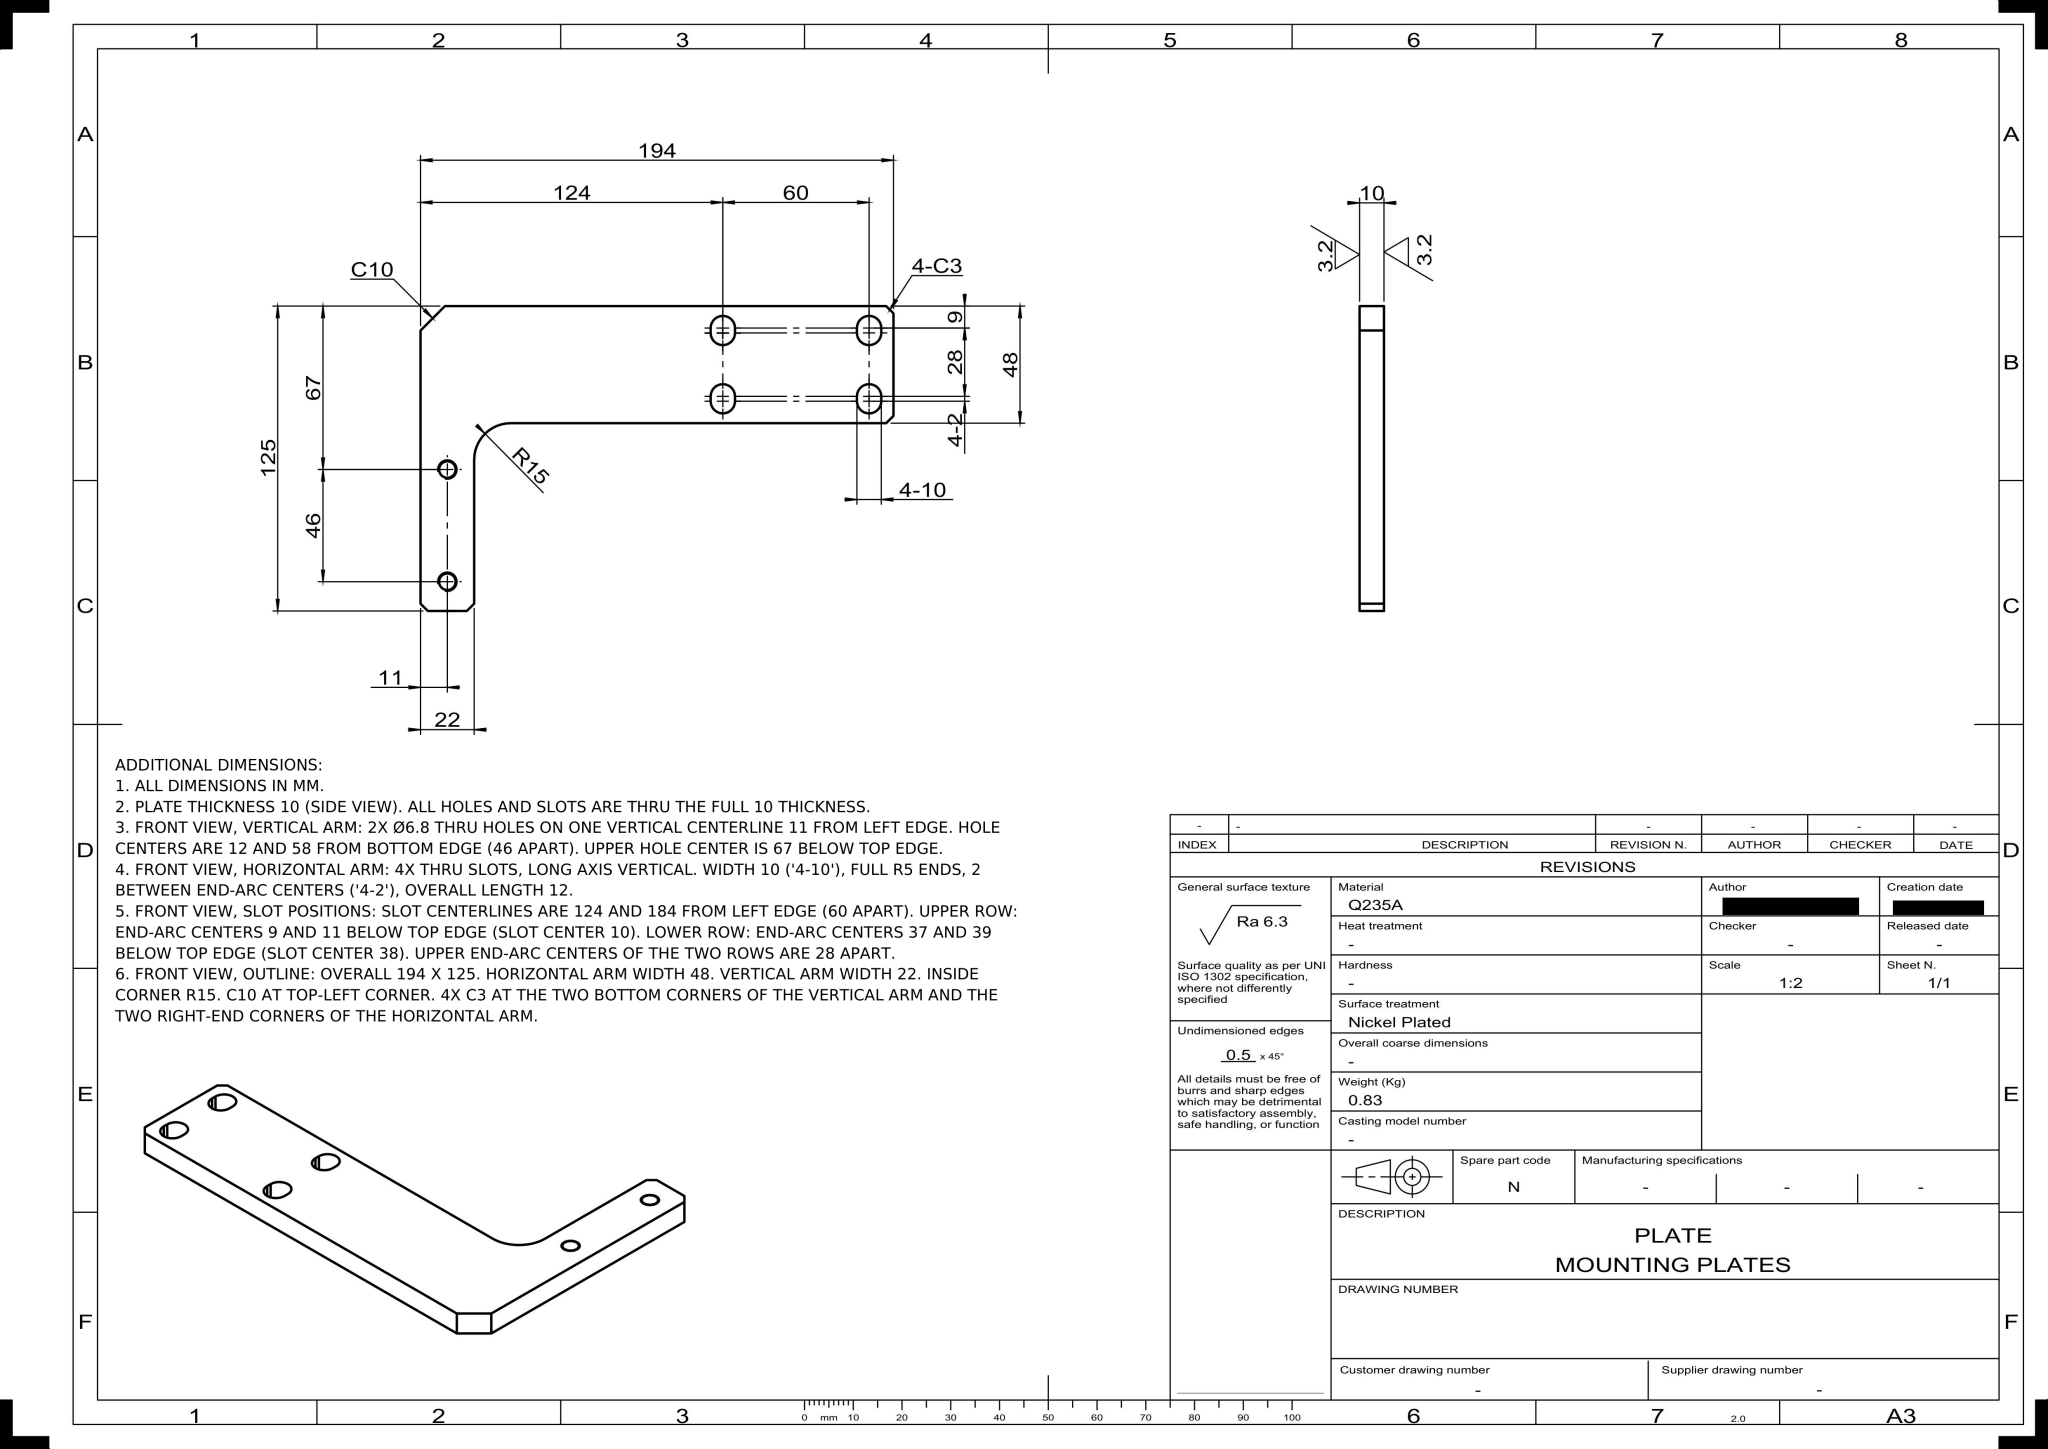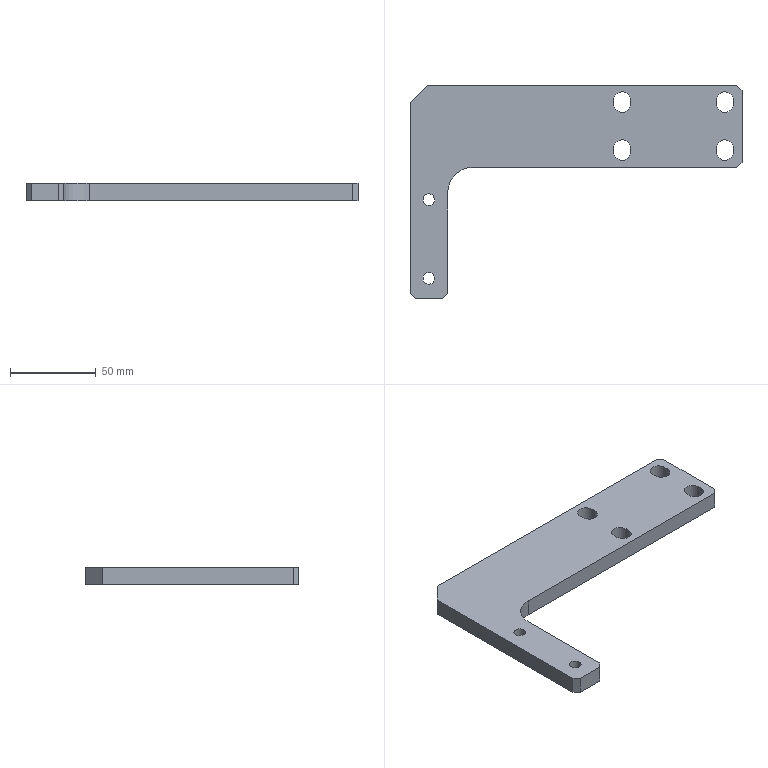Part | NX | mm | 1 solid | 32 faces | box 194 x 125 x 10 mm | volume 105195 mm3 | plane 21 | cylinder 11 | commonest cylinder face diameters 10 x8 6.8 x2 30 x1
STEP:
#1=CARTESIAN_POINT('',(0.,0.,0.));
#2=DIRECTION('',(0.,0.,1.));
#3=DIRECTION('',(1.,0.,0.));
#4=AXIS2_PLACEMENT_3D('',#1,#2,#3);
#5=(LENGTH_UNIT()NAMED_UNIT(*)SI_UNIT(.MILLI.,.METRE.));
#6=UNCERTAINTY_MEASURE_WITH_UNIT(LENGTH_MEASURE(0.00002),#5,'','');
#7=(NAMED_UNIT(*)PLANE_ANGLE_UNIT()SI_UNIT($,.RADIAN.));
#8=PLANE_ANGLE_MEASURE_WITH_UNIT(PLANE_ANGLE_MEASURE(0.01745),#7);
#9=DIMENSIONAL_EXPONENTS(0.,0.,0.,0.,0.,0.,0.);
#10=(CONVERSION_BASED_UNIT('',#8)NAMED_UNIT(#9)PLANE_ANGLE_UNIT());
#11=(NAMED_UNIT(*)SI_UNIT($,.STERADIAN.)SOLID_ANGLE_UNIT());
#12=(GEOMETRIC_REPRESENTATION_CONTEXT(3)GLOBAL_UNCERTAINTY_ASSIGNED_CONTEXT((#6))GLOBAL_UNIT_ASSIGNED_CONTEXT((#5,#10,#11))REPRESENTATION_CONTEXT('',''));
#13=SHAPE_REPRESENTATION('',(#4),#12);
#14=CARTESIAN_POINT('',(179.,-11.,0.));
#15=VERTEX_POINT('',#14);
#16=CARTESIAN_POINT('',(179.,-9.,0.));
#17=VERTEX_POINT('',#16);
#18=CARTESIAN_POINT('',(179.,-11.,0.));
#19=DIRECTION('',(0.,1.,0.));
#20=VECTOR('',#19,1.);
#21=LINE('',#18,#20);
#22=EDGE_CURVE('',#15,#17,#21,.T.);
#23=ORIENTED_EDGE('',*,*,#22,.T.);
#24=CARTESIAN_POINT('',(179.,-9.,10.));
#25=VERTEX_POINT('',#24);
#26=CARTESIAN_POINT('',(179.,-9.,10.));
#27=DIRECTION('',(0.,0.,-1.));
#28=VECTOR('',#27,1.);
#29=LINE('',#26,#28);
#30=EDGE_CURVE('',#25,#17,#29,.T.);
#31=ORIENTED_EDGE('',*,*,#30,.F.);
#32=CARTESIAN_POINT('',(179.,-11.,10.));
#33=VERTEX_POINT('',#32);
#34=CARTESIAN_POINT('',(179.,-11.,10.));
#35=DIRECTION('',(0.,1.,0.));
#36=VECTOR('',#35,1.);
#37=LINE('',#34,#36);
#38=EDGE_CURVE('',#33,#25,#37,.T.);
#39=ORIENTED_EDGE('',*,*,#38,.F.);
#40=CARTESIAN_POINT('',(179.,-11.,10.));
#41=DIRECTION('',(0.,0.,-1.));
#42=VECTOR('',#41,1.);
#43=LINE('',#40,#42);
#44=EDGE_CURVE('',#33,#15,#43,.T.);
#45=ORIENTED_EDGE('',*,*,#44,.T.);
#46=EDGE_LOOP('',(#23,#31,#39,#45));
#47=FACE_OUTER_BOUND('',#46,.T.);
#48=CARTESIAN_POINT('',(179.,-11.,10.));
#49=DIRECTION('',(-1.,0.,0.));
#50=DIRECTION('',(0.,0.,1.));
#51=AXIS2_PLACEMENT_3D('',#48,#49,#50);
#52=PLANE('',#51);
#53=ADVANCED_FACE('',(#47),#52,.F.);
#54=CARTESIAN_POINT('',(189.,-9.,0.));
#55=VERTEX_POINT('',#54);
#56=CARTESIAN_POINT('',(184.,-9.,0.));
#57=DIRECTION('',(0.,0.,-1.));
#58=DIRECTION('',(1.,0.,0.));
#59=AXIS2_PLACEMENT_3D('',#56,#57,#58);
#60=CIRCLE('',#59,5.);
#61=EDGE_CURVE('',#17,#55,#60,.T.);
#62=ORIENTED_EDGE('',*,*,#61,.T.);
#63=CARTESIAN_POINT('',(189.,-9.,10.));
#64=VERTEX_POINT('',#63);
#65=CARTESIAN_POINT('',(189.,-9.,10.));
#66=DIRECTION('',(0.,0.,-1.));
#67=VECTOR('',#66,1.);
#68=LINE('',#65,#67);
#69=EDGE_CURVE('',#64,#55,#68,.T.);
#70=ORIENTED_EDGE('',*,*,#69,.F.);
#71=CARTESIAN_POINT('',(184.,-9.,10.));
#72=DIRECTION('',(0.,0.,-1.));
#73=DIRECTION('',(1.,0.,0.));
#74=AXIS2_PLACEMENT_3D('',#71,#72,#73);
#75=CIRCLE('',#74,5.);
#76=EDGE_CURVE('',#25,#64,#75,.T.);
#77=ORIENTED_EDGE('',*,*,#76,.F.);
#78=ORIENTED_EDGE('',*,*,#30,.T.);
#79=EDGE_LOOP('',(#62,#70,#77,#78));
#80=FACE_OUTER_BOUND('',#79,.T.);
#81=CARTESIAN_POINT('',(184.,-9.,10.));
#82=DIRECTION('',(0.,0.,-1.));
#83=DIRECTION('',(-1.,0.,0.));
#84=AXIS2_PLACEMENT_3D('',#81,#82,#83);
#85=CYLINDRICAL_SURFACE('',#84,5.);
#86=ADVANCED_FACE('',(#80),#85,.F.);
#87=CARTESIAN_POINT('',(189.,-11.,0.));
#88=VERTEX_POINT('',#87);
#89=CARTESIAN_POINT('',(189.,-9.,0.));
#90=DIRECTION('',(0.,-1.,0.));
#91=VECTOR('',#90,1.);
#92=LINE('',#89,#91);
#93=EDGE_CURVE('',#55,#88,#92,.T.);
#94=ORIENTED_EDGE('',*,*,#93,.T.);
#95=CARTESIAN_POINT('',(189.,-11.,10.));
#96=VERTEX_POINT('',#95);
#97=CARTESIAN_POINT('',(189.,-11.,10.));
#98=DIRECTION('',(0.,0.,-1.));
#99=VECTOR('',#98,1.);
#100=LINE('',#97,#99);
#101=EDGE_CURVE('',#96,#88,#100,.T.);
#102=ORIENTED_EDGE('',*,*,#101,.F.);
#103=CARTESIAN_POINT('',(189.,-9.,10.));
#104=DIRECTION('',(0.,-1.,0.));
#105=VECTOR('',#104,1.);
#106=LINE('',#103,#105);
#107=EDGE_CURVE('',#64,#96,#106,.T.);
#108=ORIENTED_EDGE('',*,*,#107,.F.);
#109=ORIENTED_EDGE('',*,*,#69,.T.);
#110=EDGE_LOOP('',(#94,#102,#108,#109));
#111=FACE_OUTER_BOUND('',#110,.T.);
#112=CARTESIAN_POINT('',(189.,-9.,10.));
#113=DIRECTION('',(1.,0.,0.));
#114=DIRECTION('',(0.,0.,-1.));
#115=AXIS2_PLACEMENT_3D('',#112,#113,#114);
#116=PLANE('',#115);
#117=ADVANCED_FACE('',(#111),#116,.F.);
#118=CARTESIAN_POINT('',(179.,-39.,0.));
#119=VERTEX_POINT('',#118);
#120=CARTESIAN_POINT('',(179.,-37.,0.));
#121=VERTEX_POINT('',#120);
#122=CARTESIAN_POINT('',(179.,-39.,0.));
#123=DIRECTION('',(0.,1.,0.));
#124=VECTOR('',#123,1.);
#125=LINE('',#122,#124);
#126=EDGE_CURVE('',#119,#121,#125,.T.);
#127=ORIENTED_EDGE('',*,*,#126,.T.);
#128=CARTESIAN_POINT('',(179.,-37.,10.));
#129=VERTEX_POINT('',#128);
#130=CARTESIAN_POINT('',(179.,-37.,10.));
#131=DIRECTION('',(0.,0.,-1.));
#132=VECTOR('',#131,1.);
#133=LINE('',#130,#132);
#134=EDGE_CURVE('',#129,#121,#133,.T.);
#135=ORIENTED_EDGE('',*,*,#134,.F.);
#136=CARTESIAN_POINT('',(179.,-39.,10.));
#137=VERTEX_POINT('',#136);
#138=CARTESIAN_POINT('',(179.,-39.,10.));
#139=DIRECTION('',(0.,1.,0.));
#140=VECTOR('',#139,1.);
#141=LINE('',#138,#140);
#142=EDGE_CURVE('',#137,#129,#141,.T.);
#143=ORIENTED_EDGE('',*,*,#142,.F.);
#144=CARTESIAN_POINT('',(179.,-39.,10.));
#145=DIRECTION('',(0.,0.,-1.));
#146=VECTOR('',#145,1.);
#147=LINE('',#144,#146);
#148=EDGE_CURVE('',#137,#119,#147,.T.);
#149=ORIENTED_EDGE('',*,*,#148,.T.);
#150=EDGE_LOOP('',(#127,#135,#143,#149));
#151=FACE_OUTER_BOUND('',#150,.T.);
#152=CARTESIAN_POINT('',(179.,-39.,10.));
#153=DIRECTION('',(-1.,0.,0.));
#154=DIRECTION('',(0.,0.,1.));
#155=AXIS2_PLACEMENT_3D('',#152,#153,#154);
#156=PLANE('',#155);
#157=ADVANCED_FACE('',(#151),#156,.F.);
#158=CARTESIAN_POINT('',(189.,-37.,0.));
#159=VERTEX_POINT('',#158);
#160=CARTESIAN_POINT('',(184.,-37.,0.));
#161=DIRECTION('',(0.,0.,-1.));
#162=DIRECTION('',(1.,0.,0.));
#163=AXIS2_PLACEMENT_3D('',#160,#161,#162);
#164=CIRCLE('',#163,5.);
#165=EDGE_CURVE('',#121,#159,#164,.T.);
#166=ORIENTED_EDGE('',*,*,#165,.T.);
#167=CARTESIAN_POINT('',(189.,-37.,10.));
#168=VERTEX_POINT('',#167);
#169=CARTESIAN_POINT('',(189.,-37.,10.));
#170=DIRECTION('',(0.,0.,-1.));
#171=VECTOR('',#170,1.);
#172=LINE('',#169,#171);
#173=EDGE_CURVE('',#168,#159,#172,.T.);
#174=ORIENTED_EDGE('',*,*,#173,.F.);
#175=CARTESIAN_POINT('',(184.,-37.,10.));
#176=DIRECTION('',(0.,0.,-1.));
#177=DIRECTION('',(1.,0.,0.));
#178=AXIS2_PLACEMENT_3D('',#175,#176,#177);
#179=CIRCLE('',#178,5.);
#180=EDGE_CURVE('',#129,#168,#179,.T.);
#181=ORIENTED_EDGE('',*,*,#180,.F.);
#182=ORIENTED_EDGE('',*,*,#134,.T.);
#183=EDGE_LOOP('',(#166,#174,#181,#182));
#184=FACE_OUTER_BOUND('',#183,.T.);
#185=CARTESIAN_POINT('',(184.,-37.,10.));
#186=DIRECTION('',(0.,0.,-1.));
#187=DIRECTION('',(-1.,0.,0.));
#188=AXIS2_PLACEMENT_3D('',#185,#186,#187);
#189=CYLINDRICAL_SURFACE('',#188,5.);
#190=ADVANCED_FACE('',(#184),#189,.F.);
#191=CARTESIAN_POINT('',(189.,-39.,0.));
#192=VERTEX_POINT('',#191);
#193=CARTESIAN_POINT('',(189.,-37.,0.));
#194=DIRECTION('',(0.,-1.,0.));
#195=VECTOR('',#194,1.);
#196=LINE('',#193,#195);
#197=EDGE_CURVE('',#159,#192,#196,.T.);
#198=ORIENTED_EDGE('',*,*,#197,.T.);
#199=CARTESIAN_POINT('',(189.,-39.,10.));
#200=VERTEX_POINT('',#199);
#201=CARTESIAN_POINT('',(189.,-39.,10.));
#202=DIRECTION('',(0.,0.,-1.));
#203=VECTOR('',#202,1.);
#204=LINE('',#201,#203);
#205=EDGE_CURVE('',#200,#192,#204,.T.);
#206=ORIENTED_EDGE('',*,*,#205,.F.);
#207=CARTESIAN_POINT('',(189.,-37.,10.));
#208=DIRECTION('',(0.,-1.,0.));
#209=VECTOR('',#208,1.);
#210=LINE('',#207,#209);
#211=EDGE_CURVE('',#168,#200,#210,.T.);
#212=ORIENTED_EDGE('',*,*,#211,.F.);
#213=ORIENTED_EDGE('',*,*,#173,.T.);
#214=EDGE_LOOP('',(#198,#206,#212,#213));
#215=FACE_OUTER_BOUND('',#214,.T.);
#216=CARTESIAN_POINT('',(189.,-37.,10.));
#217=DIRECTION('',(1.,0.,0.));
#218=DIRECTION('',(0.,0.,-1.));
#219=AXIS2_PLACEMENT_3D('',#216,#217,#218);
#220=PLANE('',#219);
#221=ADVANCED_FACE('',(#215),#220,.F.);
#222=CARTESIAN_POINT('',(119.,-11.,0.));
#223=VERTEX_POINT('',#222);
#224=CARTESIAN_POINT('',(119.,-9.,0.));
#225=VERTEX_POINT('',#224);
#226=CARTESIAN_POINT('',(119.,-11.,0.));
#227=DIRECTION('',(0.,1.,0.));
#228=VECTOR('',#227,1.);
#229=LINE('',#226,#228);
#230=EDGE_CURVE('',#223,#225,#229,.T.);
#231=ORIENTED_EDGE('',*,*,#230,.T.);
#232=CARTESIAN_POINT('',(119.,-9.,10.));
#233=VERTEX_POINT('',#232);
#234=CARTESIAN_POINT('',(119.,-9.,10.));
#235=DIRECTION('',(0.,0.,-1.));
#236=VECTOR('',#235,1.);
#237=LINE('',#234,#236);
#238=EDGE_CURVE('',#233,#225,#237,.T.);
#239=ORIENTED_EDGE('',*,*,#238,.F.);
#240=CARTESIAN_POINT('',(119.,-11.,10.));
#241=VERTEX_POINT('',#240);
#242=CARTESIAN_POINT('',(119.,-11.,10.));
#243=DIRECTION('',(0.,1.,0.));
#244=VECTOR('',#243,1.);
#245=LINE('',#242,#244);
#246=EDGE_CURVE('',#241,#233,#245,.T.);
#247=ORIENTED_EDGE('',*,*,#246,.F.);
#248=CARTESIAN_POINT('',(119.,-11.,10.));
#249=DIRECTION('',(0.,0.,-1.));
#250=VECTOR('',#249,1.);
#251=LINE('',#248,#250);
#252=EDGE_CURVE('',#241,#223,#251,.T.);
#253=ORIENTED_EDGE('',*,*,#252,.T.);
#254=EDGE_LOOP('',(#231,#239,#247,#253));
#255=FACE_OUTER_BOUND('',#254,.T.);
#256=CARTESIAN_POINT('',(119.,-11.,10.));
#257=DIRECTION('',(-1.,0.,0.));
#258=DIRECTION('',(0.,0.,1.));
#259=AXIS2_PLACEMENT_3D('',#256,#257,#258);
#260=PLANE('',#259);
#261=ADVANCED_FACE('',(#255),#260,.F.);
#262=CARTESIAN_POINT('',(129.,-9.,0.));
#263=VERTEX_POINT('',#262);
#264=CARTESIAN_POINT('',(124.,-9.,0.));
#265=DIRECTION('',(0.,0.,-1.));
#266=DIRECTION('',(1.,0.,0.));
#267=AXIS2_PLACEMENT_3D('',#264,#265,#266);
#268=CIRCLE('',#267,5.);
#269=EDGE_CURVE('',#225,#263,#268,.T.);
#270=ORIENTED_EDGE('',*,*,#269,.T.);
#271=CARTESIAN_POINT('',(129.,-9.,10.));
#272=VERTEX_POINT('',#271);
#273=CARTESIAN_POINT('',(129.,-9.,10.));
#274=DIRECTION('',(0.,0.,-1.));
#275=VECTOR('',#274,1.);
#276=LINE('',#273,#275);
#277=EDGE_CURVE('',#272,#263,#276,.T.);
#278=ORIENTED_EDGE('',*,*,#277,.F.);
#279=CARTESIAN_POINT('',(124.,-9.,10.));
#280=DIRECTION('',(0.,0.,-1.));
#281=DIRECTION('',(1.,0.,0.));
#282=AXIS2_PLACEMENT_3D('',#279,#280,#281);
#283=CIRCLE('',#282,5.);
#284=EDGE_CURVE('',#233,#272,#283,.T.);
#285=ORIENTED_EDGE('',*,*,#284,.F.);
#286=ORIENTED_EDGE('',*,*,#238,.T.);
#287=EDGE_LOOP('',(#270,#278,#285,#286));
#288=FACE_OUTER_BOUND('',#287,.T.);
#289=CARTESIAN_POINT('',(124.,-9.,10.));
#290=DIRECTION('',(0.,0.,-1.));
#291=DIRECTION('',(-1.,0.,0.));
#292=AXIS2_PLACEMENT_3D('',#289,#290,#291);
#293=CYLINDRICAL_SURFACE('',#292,5.);
#294=ADVANCED_FACE('',(#288),#293,.F.);
#295=CARTESIAN_POINT('',(129.,-11.,0.));
#296=VERTEX_POINT('',#295);
#297=CARTESIAN_POINT('',(129.,-9.,0.));
#298=DIRECTION('',(0.,-1.,0.));
#299=VECTOR('',#298,1.);
#300=LINE('',#297,#299);
#301=EDGE_CURVE('',#263,#296,#300,.T.);
#302=ORIENTED_EDGE('',*,*,#301,.T.);
#303=CARTESIAN_POINT('',(129.,-11.,10.));
#304=VERTEX_POINT('',#303);
#305=CARTESIAN_POINT('',(129.,-11.,10.));
#306=DIRECTION('',(0.,0.,-1.));
#307=VECTOR('',#306,1.);
#308=LINE('',#305,#307);
#309=EDGE_CURVE('',#304,#296,#308,.T.);
#310=ORIENTED_EDGE('',*,*,#309,.F.);
#311=CARTESIAN_POINT('',(129.,-9.,10.));
#312=DIRECTION('',(0.,-1.,0.));
#313=VECTOR('',#312,1.);
#314=LINE('',#311,#313);
#315=EDGE_CURVE('',#272,#304,#314,.T.);
#316=ORIENTED_EDGE('',*,*,#315,.F.);
#317=ORIENTED_EDGE('',*,*,#277,.T.);
#318=EDGE_LOOP('',(#302,#310,#316,#317));
#319=FACE_OUTER_BOUND('',#318,.T.);
#320=CARTESIAN_POINT('',(129.,-9.,10.));
#321=DIRECTION('',(1.,0.,0.));
#322=DIRECTION('',(0.,0.,-1.));
#323=AXIS2_PLACEMENT_3D('',#320,#321,#322);
#324=PLANE('',#323);
#325=ADVANCED_FACE('',(#319),#324,.F.);
#326=CARTESIAN_POINT('',(119.,-39.,0.));
#327=VERTEX_POINT('',#326);
#328=CARTESIAN_POINT('',(119.,-37.,0.));
#329=VERTEX_POINT('',#328);
#330=CARTESIAN_POINT('',(119.,-39.,0.));
#331=DIRECTION('',(0.,1.,0.));
#332=VECTOR('',#331,1.);
#333=LINE('',#330,#332);
#334=EDGE_CURVE('',#327,#329,#333,.T.);
#335=ORIENTED_EDGE('',*,*,#334,.T.);
#336=CARTESIAN_POINT('',(119.,-37.,10.));
#337=VERTEX_POINT('',#336);
#338=CARTESIAN_POINT('',(119.,-37.,10.));
#339=DIRECTION('',(0.,0.,-1.));
#340=VECTOR('',#339,1.);
#341=LINE('',#338,#340);
#342=EDGE_CURVE('',#337,#329,#341,.T.);
#343=ORIENTED_EDGE('',*,*,#342,.F.);
#344=CARTESIAN_POINT('',(119.,-39.,10.));
#345=VERTEX_POINT('',#344);
#346=CARTESIAN_POINT('',(119.,-39.,10.));
#347=DIRECTION('',(0.,1.,0.));
#348=VECTOR('',#347,1.);
#349=LINE('',#346,#348);
#350=EDGE_CURVE('',#345,#337,#349,.T.);
#351=ORIENTED_EDGE('',*,*,#350,.F.);
#352=CARTESIAN_POINT('',(119.,-39.,10.));
#353=DIRECTION('',(0.,0.,-1.));
#354=VECTOR('',#353,1.);
#355=LINE('',#352,#354);
#356=EDGE_CURVE('',#345,#327,#355,.T.);
#357=ORIENTED_EDGE('',*,*,#356,.T.);
#358=EDGE_LOOP('',(#335,#343,#351,#357));
#359=FACE_OUTER_BOUND('',#358,.T.);
#360=CARTESIAN_POINT('',(119.,-39.,10.));
#361=DIRECTION('',(-1.,0.,0.));
#362=DIRECTION('',(0.,0.,1.));
#363=AXIS2_PLACEMENT_3D('',#360,#361,#362);
#364=PLANE('',#363);
#365=ADVANCED_FACE('',(#359),#364,.F.);
#366=CARTESIAN_POINT('',(129.,-37.,0.));
#367=VERTEX_POINT('',#366);
#368=CARTESIAN_POINT('',(124.,-37.,0.));
#369=DIRECTION('',(0.,0.,-1.));
#370=DIRECTION('',(1.,0.,0.));
#371=AXIS2_PLACEMENT_3D('',#368,#369,#370);
#372=CIRCLE('',#371,5.);
#373=EDGE_CURVE('',#329,#367,#372,.T.);
#374=ORIENTED_EDGE('',*,*,#373,.T.);
#375=CARTESIAN_POINT('',(129.,-37.,10.));
#376=VERTEX_POINT('',#375);
#377=CARTESIAN_POINT('',(129.,-37.,10.));
#378=DIRECTION('',(0.,0.,-1.));
#379=VECTOR('',#378,1.);
#380=LINE('',#377,#379);
#381=EDGE_CURVE('',#376,#367,#380,.T.);
#382=ORIENTED_EDGE('',*,*,#381,.F.);
#383=CARTESIAN_POINT('',(124.,-37.,10.));
#384=DIRECTION('',(0.,0.,-1.));
#385=DIRECTION('',(1.,0.,0.));
#386=AXIS2_PLACEMENT_3D('',#383,#384,#385);
#387=CIRCLE('',#386,5.);
#388=EDGE_CURVE('',#337,#376,#387,.T.);
#389=ORIENTED_EDGE('',*,*,#388,.F.);
#390=ORIENTED_EDGE('',*,*,#342,.T.);
#391=EDGE_LOOP('',(#374,#382,#389,#390));
#392=FACE_OUTER_BOUND('',#391,.T.);
#393=CARTESIAN_POINT('',(124.,-37.,10.));
#394=DIRECTION('',(0.,0.,-1.));
#395=DIRECTION('',(-1.,0.,0.));
#396=AXIS2_PLACEMENT_3D('',#393,#394,#395);
#397=CYLINDRICAL_SURFACE('',#396,5.);
#398=ADVANCED_FACE('',(#392),#397,.F.);
#399=CARTESIAN_POINT('',(129.,-39.,0.));
#400=VERTEX_POINT('',#399);
#401=CARTESIAN_POINT('',(129.,-37.,0.));
#402=DIRECTION('',(0.,-1.,0.));
#403=VECTOR('',#402,1.);
#404=LINE('',#401,#403);
#405=EDGE_CURVE('',#367,#400,#404,.T.);
#406=ORIENTED_EDGE('',*,*,#405,.T.);
#407=CARTESIAN_POINT('',(129.,-39.,10.));
#408=VERTEX_POINT('',#407);
#409=CARTESIAN_POINT('',(129.,-39.,10.));
#410=DIRECTION('',(0.,0.,-1.));
#411=VECTOR('',#410,1.);
#412=LINE('',#409,#411);
#413=EDGE_CURVE('',#408,#400,#412,.T.);
#414=ORIENTED_EDGE('',*,*,#413,.F.);
#415=CARTESIAN_POINT('',(129.,-37.,10.));
#416=DIRECTION('',(0.,-1.,0.));
#417=VECTOR('',#416,1.);
#418=LINE('',#415,#417);
#419=EDGE_CURVE('',#376,#408,#418,.T.);
#420=ORIENTED_EDGE('',*,*,#419,.F.);
#421=ORIENTED_EDGE('',*,*,#381,.T.);
#422=EDGE_LOOP('',(#406,#414,#420,#421));
#423=FACE_OUTER_BOUND('',#422,.T.);
#424=CARTESIAN_POINT('',(129.,-37.,10.));
#425=DIRECTION('',(1.,0.,0.));
#426=DIRECTION('',(0.,0.,-1.));
#427=AXIS2_PLACEMENT_3D('',#424,#425,#426);
#428=PLANE('',#427);
#429=ADVANCED_FACE('',(#423),#428,.F.);
#430=CARTESIAN_POINT('',(0.,-10.,0.));
#431=VERTEX_POINT('',#430);
#432=CARTESIAN_POINT('',(0.,-122.,0.));
#433=VERTEX_POINT('',#432);
#434=CARTESIAN_POINT('',(0.,0.,0.));
#435=DIRECTION('',(0.,-1.,0.));
#436=VECTOR('',#435,1.);
#437=LINE('',#434,#436);
#438=EDGE_CURVE('',#431,#433,#437,.T.);
#439=ORIENTED_EDGE('',*,*,#438,.T.);
#440=CARTESIAN_POINT('',(0.,-122.,10.));
#441=VERTEX_POINT('',#440);
#442=CARTESIAN_POINT('',(0.,-122.,10.));
#443=DIRECTION('',(0.,0.,1.));
#444=VECTOR('',#443,1.);
#445=LINE('',#442,#444);
#446=EDGE_CURVE('',#433,#441,#445,.T.);
#447=ORIENTED_EDGE('',*,*,#446,.T.);
#448=CARTESIAN_POINT('',(0.,-10.,10.));
#449=VERTEX_POINT('',#448);
#450=CARTESIAN_POINT('',(0.,0.,10.));
#451=DIRECTION('',(0.,-1.,0.));
#452=VECTOR('',#451,1.);
#453=LINE('',#450,#452);
#454=EDGE_CURVE('',#449,#441,#453,.T.);
#455=ORIENTED_EDGE('',*,*,#454,.F.);
#456=CARTESIAN_POINT('',(0.,-10.,10.));
#457=DIRECTION('',(0.,0.,-1.));
#458=VECTOR('',#457,1.);
#459=LINE('',#456,#458);
#460=EDGE_CURVE('',#449,#431,#459,.T.);
#461=ORIENTED_EDGE('',*,*,#460,.T.);
#462=EDGE_LOOP('',(#439,#447,#455,#461));
#463=FACE_OUTER_BOUND('',#462,.T.);
#464=CARTESIAN_POINT('',(0.,0.,10.));
#465=DIRECTION('',(1.,0.,0.));
#466=DIRECTION('',(0.,0.,-1.));
#467=AXIS2_PLACEMENT_3D('',#464,#465,#466);
#468=PLANE('',#467);
#469=ADVANCED_FACE('',(#463),#468,.F.);
#470=CARTESIAN_POINT('',(3.,-125.,0.));
#471=VERTEX_POINT('',#470);
#472=CARTESIAN_POINT('',(19.,-125.,0.));
#473=VERTEX_POINT('',#472);
#474=CARTESIAN_POINT('',(-0.,-125.,0.));
#475=DIRECTION('',(1.,0.,0.));
#476=VECTOR('',#475,1.);
#477=LINE('',#474,#476);
#478=EDGE_CURVE('',#471,#473,#477,.T.);
#479=ORIENTED_EDGE('',*,*,#478,.T.);
#480=CARTESIAN_POINT('',(19.,-125.,10.));
#481=VERTEX_POINT('',#480);
#482=CARTESIAN_POINT('',(19.,-125.,10.));
#483=DIRECTION('',(0.,0.,1.));
#484=VECTOR('',#483,1.);
#485=LINE('',#482,#484);
#486=EDGE_CURVE('',#473,#481,#485,.T.);
#487=ORIENTED_EDGE('',*,*,#486,.T.);
#488=CARTESIAN_POINT('',(3.,-125.,10.));
#489=VERTEX_POINT('',#488);
#490=CARTESIAN_POINT('',(-0.,-125.,10.));
#491=DIRECTION('',(1.,0.,0.));
#492=VECTOR('',#491,1.);
#493=LINE('',#490,#492);
#494=EDGE_CURVE('',#489,#481,#493,.T.);
#495=ORIENTED_EDGE('',*,*,#494,.F.);
#496=CARTESIAN_POINT('',(3.,-125.,10.));
#497=DIRECTION('',(0.,0.,-1.));
#498=VECTOR('',#497,1.);
#499=LINE('',#496,#498);
#500=EDGE_CURVE('',#489,#471,#499,.T.);
#501=ORIENTED_EDGE('',*,*,#500,.T.);
#502=EDGE_LOOP('',(#479,#487,#495,#501));
#503=FACE_OUTER_BOUND('',#502,.T.);
#504=CARTESIAN_POINT('',(-0.,-125.,10.));
#505=DIRECTION('',(0.,1.,0.));
#506=DIRECTION('',(0.,0.,1.));
#507=AXIS2_PLACEMENT_3D('',#504,#505,#506);
#508=PLANE('',#507);
#509=ADVANCED_FACE('',(#503),#508,.F.);
#510=CARTESIAN_POINT('',(22.,-122.,0.));
#511=VERTEX_POINT('',#510);
#512=CARTESIAN_POINT('',(22.,-63.,0.));
#513=VERTEX_POINT('',#512);
#514=CARTESIAN_POINT('',(22.,-125.,0.));
#515=DIRECTION('',(0.,1.,0.));
#516=VECTOR('',#515,1.);
#517=LINE('',#514,#516);
#518=EDGE_CURVE('',#511,#513,#517,.T.);
#519=ORIENTED_EDGE('',*,*,#518,.T.);
#520=CARTESIAN_POINT('',(22.,-63.,10.));
#521=VERTEX_POINT('',#520);
#522=CARTESIAN_POINT('',(22.,-63.,10.));
#523=DIRECTION('',(0.,0.,1.));
#524=VECTOR('',#523,1.);
#525=LINE('',#522,#524);
#526=EDGE_CURVE('',#513,#521,#525,.T.);
#527=ORIENTED_EDGE('',*,*,#526,.T.);
#528=CARTESIAN_POINT('',(22.,-122.,10.));
#529=VERTEX_POINT('',#528);
#530=CARTESIAN_POINT('',(22.,-125.,10.));
#531=DIRECTION('',(0.,1.,0.));
#532=VECTOR('',#531,1.);
#533=LINE('',#530,#532);
#534=EDGE_CURVE('',#529,#521,#533,.T.);
#535=ORIENTED_EDGE('',*,*,#534,.F.);
#536=CARTESIAN_POINT('',(22.,-122.,10.));
#537=DIRECTION('',(0.,0.,-1.));
#538=VECTOR('',#537,1.);
#539=LINE('',#536,#538);
#540=EDGE_CURVE('',#529,#511,#539,.T.);
#541=ORIENTED_EDGE('',*,*,#540,.T.);
#542=EDGE_LOOP('',(#519,#527,#535,#541));
#543=FACE_OUTER_BOUND('',#542,.T.);
#544=CARTESIAN_POINT('',(22.,-125.,10.));
#545=DIRECTION('',(-1.,0.,0.));
#546=DIRECTION('',(-0.,-1.,0.));
#547=AXIS2_PLACEMENT_3D('',#544,#545,#546);
#548=PLANE('',#547);
#549=ADVANCED_FACE('',(#543),#548,.F.);
#550=CARTESIAN_POINT('',(37.,-48.,10.));
#551=VERTEX_POINT('',#550);
#552=CARTESIAN_POINT('',(191.,-48.,10.));
#553=VERTEX_POINT('',#552);
#554=CARTESIAN_POINT('',(22.,-48.,10.));
#555=DIRECTION('',(1.,0.,0.));
#556=VECTOR('',#555,1.);
#557=LINE('',#554,#556);
#558=EDGE_CURVE('',#551,#553,#557,.T.);
#559=ORIENTED_EDGE('',*,*,#558,.F.);
#560=CARTESIAN_POINT('',(37.,-48.,0.));
#561=VERTEX_POINT('',#560);
#562=CARTESIAN_POINT('',(37.,-48.,0.));
#563=DIRECTION('',(0.,0.,-1.));
#564=VECTOR('',#563,1.);
#565=LINE('',#562,#564);
#566=EDGE_CURVE('',#551,#561,#565,.T.);
#567=ORIENTED_EDGE('',*,*,#566,.T.);
#568=CARTESIAN_POINT('',(191.,-48.,0.));
#569=VERTEX_POINT('',#568);
#570=CARTESIAN_POINT('',(22.,-48.,0.));
#571=DIRECTION('',(1.,0.,0.));
#572=VECTOR('',#571,1.);
#573=LINE('',#570,#572);
#574=EDGE_CURVE('',#561,#569,#573,.T.);
#575=ORIENTED_EDGE('',*,*,#574,.T.);
#576=CARTESIAN_POINT('',(191.,-48.,10.));
#577=DIRECTION('',(0.,0.,1.));
#578=VECTOR('',#577,1.);
#579=LINE('',#576,#578);
#580=EDGE_CURVE('',#569,#553,#579,.T.);
#581=ORIENTED_EDGE('',*,*,#580,.T.);
#582=EDGE_LOOP('',(#559,#567,#575,#581));
#583=FACE_OUTER_BOUND('',#582,.T.);
#584=CARTESIAN_POINT('',(22.,-48.,10.));
#585=DIRECTION('',(0.,1.,0.));
#586=DIRECTION('',(0.,0.,1.));
#587=AXIS2_PLACEMENT_3D('',#584,#585,#586);
#588=PLANE('',#587);
#589=ADVANCED_FACE('',(#583),#588,.F.);
#590=CARTESIAN_POINT('',(194.,-45.,10.));
#591=VERTEX_POINT('',#590);
#592=CARTESIAN_POINT('',(194.,-3.,10.));
#593=VERTEX_POINT('',#592);
#594=CARTESIAN_POINT('',(194.,-48.,10.));
#595=DIRECTION('',(0.,1.,0.));
#596=VECTOR('',#595,1.);
#597=LINE('',#594,#596);
#598=EDGE_CURVE('',#591,#593,#597,.T.);
#599=ORIENTED_EDGE('',*,*,#598,.F.);
#600=CARTESIAN_POINT('',(194.,-45.,0.));
#601=VERTEX_POINT('',#600);
#602=CARTESIAN_POINT('',(194.,-45.,10.));
#603=DIRECTION('',(0.,0.,-1.));
#604=VECTOR('',#603,1.);
#605=LINE('',#602,#604);
#606=EDGE_CURVE('',#591,#601,#605,.T.);
#607=ORIENTED_EDGE('',*,*,#606,.T.);
#608=CARTESIAN_POINT('',(194.,-3.,0.));
#609=VERTEX_POINT('',#608);
#610=CARTESIAN_POINT('',(194.,-48.,0.));
#611=DIRECTION('',(0.,1.,0.));
#612=VECTOR('',#611,1.);
#613=LINE('',#610,#612);
#614=EDGE_CURVE('',#601,#609,#613,.T.);
#615=ORIENTED_EDGE('',*,*,#614,.T.);
#616=CARTESIAN_POINT('',(194.,-3.,10.));
#617=DIRECTION('',(0.,0.,1.));
#618=VECTOR('',#617,1.);
#619=LINE('',#616,#618);
#620=EDGE_CURVE('',#609,#593,#619,.T.);
#621=ORIENTED_EDGE('',*,*,#620,.T.);
#622=EDGE_LOOP('',(#599,#607,#615,#621));
#623=FACE_OUTER_BOUND('',#622,.T.);
#624=CARTESIAN_POINT('',(194.,-48.,10.));
#625=DIRECTION('',(-1.,0.,0.));
#626=DIRECTION('',(0.,0.,1.));
#627=AXIS2_PLACEMENT_3D('',#624,#625,#626);
#628=PLANE('',#627);
#629=ADVANCED_FACE('',(#623),#628,.F.);
#630=CARTESIAN_POINT('',(184.,-39.,0.));
#631=DIRECTION('',(0.,0.,-1.));
#632=DIRECTION('',(1.,0.,0.));
#633=AXIS2_PLACEMENT_3D('',#630,#631,#632);
#634=CIRCLE('',#633,5.);
#635=EDGE_CURVE('',#192,#119,#634,.T.);
#636=ORIENTED_EDGE('',*,*,#635,.T.);
#637=ORIENTED_EDGE('',*,*,#148,.F.);
#638=CARTESIAN_POINT('',(184.,-39.,10.));
#639=DIRECTION('',(0.,0.,-1.));
#640=DIRECTION('',(1.,0.,0.));
#641=AXIS2_PLACEMENT_3D('',#638,#639,#640);
#642=CIRCLE('',#641,5.);
#643=EDGE_CURVE('',#200,#137,#642,.T.);
#644=ORIENTED_EDGE('',*,*,#643,.F.);
#645=ORIENTED_EDGE('',*,*,#205,.T.);
#646=EDGE_LOOP('',(#636,#637,#644,#645));
#647=FACE_OUTER_BOUND('',#646,.T.);
#648=CARTESIAN_POINT('',(184.,-39.,10.));
#649=DIRECTION('',(0.,0.,-1.));
#650=DIRECTION('',(-1.,0.,0.));
#651=AXIS2_PLACEMENT_3D('',#648,#649,#650);
#652=CYLINDRICAL_SURFACE('',#651,5.);
#653=ADVANCED_FACE('',(#647),#652,.F.);
#654=CARTESIAN_POINT('',(124.,-11.,0.));
#655=DIRECTION('',(0.,0.,-1.));
#656=DIRECTION('',(1.,0.,0.));
#657=AXIS2_PLACEMENT_3D('',#654,#655,#656);
#658=CIRCLE('',#657,5.);
#659=EDGE_CURVE('',#296,#223,#658,.T.);
#660=ORIENTED_EDGE('',*,*,#659,.T.);
#661=ORIENTED_EDGE('',*,*,#252,.F.);
#662=CARTESIAN_POINT('',(124.,-11.,10.));
#663=DIRECTION('',(0.,0.,-1.));
#664=DIRECTION('',(1.,0.,0.));
#665=AXIS2_PLACEMENT_3D('',#662,#663,#664);
#666=CIRCLE('',#665,5.);
#667=EDGE_CURVE('',#304,#241,#666,.T.);
#668=ORIENTED_EDGE('',*,*,#667,.F.);
#669=ORIENTED_EDGE('',*,*,#309,.T.);
#670=EDGE_LOOP('',(#660,#661,#668,#669));
#671=FACE_OUTER_BOUND('',#670,.T.);
#672=CARTESIAN_POINT('',(124.,-11.,10.));
#673=DIRECTION('',(0.,0.,-1.));
#674=DIRECTION('',(-1.,0.,0.));
#675=AXIS2_PLACEMENT_3D('',#672,#673,#674);
#676=CYLINDRICAL_SURFACE('',#675,5.);
#677=ADVANCED_FACE('',(#671),#676,.F.);
#678=CARTESIAN_POINT('',(124.,-39.,0.));
#679=DIRECTION('',(0.,0.,-1.));
#680=DIRECTION('',(1.,0.,0.));
#681=AXIS2_PLACEMENT_3D('',#678,#679,#680);
#682=CIRCLE('',#681,5.);
#683=EDGE_CURVE('',#400,#327,#682,.T.);
#684=ORIENTED_EDGE('',*,*,#683,.T.);
#685=ORIENTED_EDGE('',*,*,#356,.F.);
#686=CARTESIAN_POINT('',(124.,-39.,10.));
#687=DIRECTION('',(0.,0.,-1.));
#688=DIRECTION('',(1.,0.,0.));
#689=AXIS2_PLACEMENT_3D('',#686,#687,#688);
#690=CIRCLE('',#689,5.);
#691=EDGE_CURVE('',#408,#345,#690,.T.);
#692=ORIENTED_EDGE('',*,*,#691,.F.);
#693=ORIENTED_EDGE('',*,*,#413,.T.);
#694=EDGE_LOOP('',(#684,#685,#692,#693));
#695=FACE_OUTER_BOUND('',#694,.T.);
#696=CARTESIAN_POINT('',(124.,-39.,10.));
#697=DIRECTION('',(0.,0.,-1.));
#698=DIRECTION('',(-1.,0.,0.));
#699=AXIS2_PLACEMENT_3D('',#696,#697,#698);
#700=CYLINDRICAL_SURFACE('',#699,5.);
#701=ADVANCED_FACE('',(#695),#700,.F.);
#702=CARTESIAN_POINT('',(191.,0.,10.));
#703=VERTEX_POINT('',#702);
#704=CARTESIAN_POINT('',(10.,0.,10.));
#705=VERTEX_POINT('',#704);
#706=CARTESIAN_POINT('',(194.,0.,10.));
#707=DIRECTION('',(-1.,0.,0.));
#708=VECTOR('',#707,1.);
#709=LINE('',#706,#708);
#710=EDGE_CURVE('',#703,#705,#709,.T.);
#711=ORIENTED_EDGE('',*,*,#710,.F.);
#712=CARTESIAN_POINT('',(191.,0.,0.));
#713=VERTEX_POINT('',#712);
#714=CARTESIAN_POINT('',(191.,0.,10.));
#715=DIRECTION('',(0.,0.,-1.));
#716=VECTOR('',#715,1.);
#717=LINE('',#714,#716);
#718=EDGE_CURVE('',#703,#713,#717,.T.);
#719=ORIENTED_EDGE('',*,*,#718,.T.);
#720=CARTESIAN_POINT('',(10.,0.,0.));
#721=VERTEX_POINT('',#720);
#722=CARTESIAN_POINT('',(194.,0.,0.));
#723=DIRECTION('',(-1.,0.,0.));
#724=VECTOR('',#723,1.);
#725=LINE('',#722,#724);
#726=EDGE_CURVE('',#713,#721,#725,.T.);
#727=ORIENTED_EDGE('',*,*,#726,.T.);
#728=CARTESIAN_POINT('',(10.,0.,10.));
#729=DIRECTION('',(0.,0.,1.));
#730=VECTOR('',#729,1.);
#731=LINE('',#728,#730);
#732=EDGE_CURVE('',#721,#705,#731,.T.);
#733=ORIENTED_EDGE('',*,*,#732,.T.);
#734=EDGE_LOOP('',(#711,#719,#727,#733));
#735=FACE_OUTER_BOUND('',#734,.T.);
#736=CARTESIAN_POINT('',(194.,0.,10.));
#737=DIRECTION('',(0.,-1.,0.));
#738=DIRECTION('',(0.,0.,-1.));
#739=AXIS2_PLACEMENT_3D('',#736,#737,#738);
#740=PLANE('',#739);
#741=ADVANCED_FACE('',(#735),#740,.F.);
#742=CARTESIAN_POINT('',(184.,-11.,0.));
#743=DIRECTION('',(0.,0.,-1.));
#744=DIRECTION('',(1.,0.,0.));
#745=AXIS2_PLACEMENT_3D('',#742,#743,#744);
#746=CIRCLE('',#745,5.);
#747=EDGE_CURVE('',#88,#15,#746,.T.);
#748=ORIENTED_EDGE('',*,*,#747,.T.);
#749=ORIENTED_EDGE('',*,*,#44,.F.);
#750=CARTESIAN_POINT('',(184.,-11.,10.));
#751=DIRECTION('',(0.,0.,-1.));
#752=DIRECTION('',(1.,0.,0.));
#753=AXIS2_PLACEMENT_3D('',#750,#751,#752);
#754=CIRCLE('',#753,5.);
#755=EDGE_CURVE('',#96,#33,#754,.T.);
#756=ORIENTED_EDGE('',*,*,#755,.F.);
#757=ORIENTED_EDGE('',*,*,#101,.T.);
#758=EDGE_LOOP('',(#748,#749,#756,#757));
#759=FACE_OUTER_BOUND('',#758,.T.);
#760=CARTESIAN_POINT('',(184.,-11.,10.));
#761=DIRECTION('',(0.,0.,-1.));
#762=DIRECTION('',(-1.,0.,0.));
#763=AXIS2_PLACEMENT_3D('',#760,#761,#762);
#764=CYLINDRICAL_SURFACE('',#763,5.);
#765=ADVANCED_FACE('',(#759),#764,.F.);
#766=CARTESIAN_POINT('',(7.6,-67.,10.));
#767=VERTEX_POINT('',#766);
#768=CARTESIAN_POINT('',(11.,-67.,10.));
#769=DIRECTION('',(0.,0.,-1.));
#770=DIRECTION('',(-1.,0.,0.));
#771=AXIS2_PLACEMENT_3D('',#768,#769,#770);
#772=CIRCLE('',#771,3.4);
#773=EDGE_CURVE('',#767,#767,#772,.T.);
#774=ORIENTED_EDGE('',*,*,#773,.T.);
#775=EDGE_LOOP('',(#774));
#776=FACE_BOUND('',#775,.T.);
#777=CARTESIAN_POINT('',(7.6,-113.,10.));
#778=VERTEX_POINT('',#777);
#779=CARTESIAN_POINT('',(11.,-113.,10.));
#780=DIRECTION('',(0.,0.,-1.));
#781=DIRECTION('',(-1.,0.,0.));
#782=AXIS2_PLACEMENT_3D('',#779,#780,#781);
#783=CIRCLE('',#782,3.4);
#784=EDGE_CURVE('',#778,#778,#783,.T.);
#785=ORIENTED_EDGE('',*,*,#784,.T.);
#786=EDGE_LOOP('',(#785));
#787=FACE_BOUND('',#786,.T.);
#788=ORIENTED_EDGE('',*,*,#494,.T.);
#789=CARTESIAN_POINT('',(22.,-122.,10.));
#790=DIRECTION('',(0.7071,0.7071,0.));
#791=VECTOR('',#790,1.);
#792=LINE('',#789,#791);
#793=EDGE_CURVE('',#481,#529,#792,.T.);
#794=ORIENTED_EDGE('',*,*,#793,.T.);
#795=ORIENTED_EDGE('',*,*,#534,.T.);
#796=CARTESIAN_POINT('',(37.,-63.,10.));
#797=DIRECTION('',(0.,0.,-1.));
#798=DIRECTION('',(-1.,0.,0.));
#799=AXIS2_PLACEMENT_3D('',#796,#797,#798);
#800=CIRCLE('',#799,15.);
#801=EDGE_CURVE('',#521,#551,#800,.T.);
#802=ORIENTED_EDGE('',*,*,#801,.T.);
#803=ORIENTED_EDGE('',*,*,#558,.T.);
#804=CARTESIAN_POINT('',(194.,-45.,10.));
#805=DIRECTION('',(0.7071,0.7071,0.));
#806=VECTOR('',#805,1.);
#807=LINE('',#804,#806);
#808=EDGE_CURVE('',#553,#591,#807,.T.);
#809=ORIENTED_EDGE('',*,*,#808,.T.);
#810=ORIENTED_EDGE('',*,*,#598,.T.);
#811=CARTESIAN_POINT('',(191.,0.,10.));
#812=DIRECTION('',(-0.7071,0.7071,0.));
#813=VECTOR('',#812,1.);
#814=LINE('',#811,#813);
#815=EDGE_CURVE('',#593,#703,#814,.T.);
#816=ORIENTED_EDGE('',*,*,#815,.T.);
#817=ORIENTED_EDGE('',*,*,#710,.T.);
#818=CARTESIAN_POINT('',(0.,-10.,10.));
#819=DIRECTION('',(-0.7071,-0.7071,0.));
#820=VECTOR('',#819,1.);
#821=LINE('',#818,#820);
#822=EDGE_CURVE('',#705,#449,#821,.T.);
#823=ORIENTED_EDGE('',*,*,#822,.T.);
#824=ORIENTED_EDGE('',*,*,#454,.T.);
#825=CARTESIAN_POINT('',(3.,-125.,10.));
#826=DIRECTION('',(0.7071,-0.7071,0.));
#827=VECTOR('',#826,1.);
#828=LINE('',#825,#827);
#829=EDGE_CURVE('',#441,#489,#828,.T.);
#830=ORIENTED_EDGE('',*,*,#829,.T.);
#831=EDGE_LOOP('',(#788,#794,#795,#802,#803,#809,#810,#816,#817,#823,#824,#830));
#832=FACE_BOUND('',#831,.T.);
#833=ORIENTED_EDGE('',*,*,#350,.T.);
#834=ORIENTED_EDGE('',*,*,#388,.T.);
#835=ORIENTED_EDGE('',*,*,#419,.T.);
#836=ORIENTED_EDGE('',*,*,#691,.T.);
#837=EDGE_LOOP('',(#833,#834,#835,#836));
#838=FACE_BOUND('',#837,.T.);
#839=ORIENTED_EDGE('',*,*,#246,.T.);
#840=ORIENTED_EDGE('',*,*,#284,.T.);
#841=ORIENTED_EDGE('',*,*,#315,.T.);
#842=ORIENTED_EDGE('',*,*,#667,.T.);
#843=EDGE_LOOP('',(#839,#840,#841,#842));
#844=FACE_BOUND('',#843,.T.);
#845=ORIENTED_EDGE('',*,*,#142,.T.);
#846=ORIENTED_EDGE('',*,*,#180,.T.);
#847=ORIENTED_EDGE('',*,*,#211,.T.);
#848=ORIENTED_EDGE('',*,*,#643,.T.);
#849=EDGE_LOOP('',(#845,#846,#847,#848));
#850=FACE_BOUND('',#849,.T.);
#851=ORIENTED_EDGE('',*,*,#38,.T.);
#852=ORIENTED_EDGE('',*,*,#76,.T.);
#853=ORIENTED_EDGE('',*,*,#107,.T.);
#854=ORIENTED_EDGE('',*,*,#755,.T.);
#855=EDGE_LOOP('',(#851,#852,#853,#854));
#856=FACE_BOUND('',#855,.T.);
#857=CARTESIAN_POINT('',(124.,-37.,10.));
#858=DIRECTION('',(0.,0.,-1.));
#859=DIRECTION('',(-1.,0.,0.));
#860=AXIS2_PLACEMENT_3D('',#857,#858,#859);
#861=PLANE('',#860);
#862=ADVANCED_FACE('',(#776,#787,#832,#838,#844,#850,#856),#861,.F.);
#863=CARTESIAN_POINT('',(14.4,-67.,0.));
#864=VERTEX_POINT('',#863);
#865=CARTESIAN_POINT('',(11.,-67.,0.));
#866=DIRECTION('',(0.,0.,1.));
#867=DIRECTION('',(1.,0.,0.));
#868=AXIS2_PLACEMENT_3D('',#865,#866,#867);
#869=CIRCLE('',#868,3.4);
#870=EDGE_CURVE('',#864,#864,#869,.T.);
#871=ORIENTED_EDGE('',*,*,#870,.T.);
#872=EDGE_LOOP('',(#871));
#873=FACE_BOUND('',#872,.T.);
#874=CARTESIAN_POINT('',(14.4,-113.,0.));
#875=VERTEX_POINT('',#874);
#876=CARTESIAN_POINT('',(11.,-113.,0.));
#877=DIRECTION('',(0.,0.,1.));
#878=DIRECTION('',(1.,0.,0.));
#879=AXIS2_PLACEMENT_3D('',#876,#877,#878);
#880=CIRCLE('',#879,3.4);
#881=EDGE_CURVE('',#875,#875,#880,.T.);
#882=ORIENTED_EDGE('',*,*,#881,.T.);
#883=EDGE_LOOP('',(#882));
#884=FACE_BOUND('',#883,.T.);
#885=ORIENTED_EDGE('',*,*,#518,.F.);
#886=CARTESIAN_POINT('',(115.5,-28.5,0.));
#887=DIRECTION('',(-0.7071,-0.7071,0.));
#888=VECTOR('',#887,1.);
#889=LINE('',#886,#888);
#890=EDGE_CURVE('',#511,#473,#889,.T.);
#891=ORIENTED_EDGE('',*,*,#890,.T.);
#892=ORIENTED_EDGE('',*,*,#478,.F.);
#893=CARTESIAN_POINT('',(19.5,-141.5,0.));
#894=DIRECTION('',(-0.7071,0.7071,0.));
#895=VECTOR('',#894,1.);
#896=LINE('',#893,#895);
#897=EDGE_CURVE('',#471,#433,#896,.T.);
#898=ORIENTED_EDGE('',*,*,#897,.T.);
#899=ORIENTED_EDGE('',*,*,#438,.F.);
#900=CARTESIAN_POINT('',(48.5,38.5,0.));
#901=DIRECTION('',(0.7071,0.7071,0.));
#902=VECTOR('',#901,1.);
#903=LINE('',#900,#902);
#904=EDGE_CURVE('',#431,#721,#903,.T.);
#905=ORIENTED_EDGE('',*,*,#904,.T.);
#906=ORIENTED_EDGE('',*,*,#726,.F.);
#907=CARTESIAN_POINT('',(176.,15.,0.));
#908=DIRECTION('',(0.7071,-0.7071,0.));
#909=VECTOR('',#908,1.);
#910=LINE('',#907,#909);
#911=EDGE_CURVE('',#713,#609,#910,.T.);
#912=ORIENTED_EDGE('',*,*,#911,.T.);
#913=ORIENTED_EDGE('',*,*,#614,.F.);
#914=CARTESIAN_POINT('',(163.,-76.,0.));
#915=DIRECTION('',(-0.7071,-0.7071,0.));
#916=VECTOR('',#915,1.);
#917=LINE('',#914,#916);
#918=EDGE_CURVE('',#601,#569,#917,.T.);
#919=ORIENTED_EDGE('',*,*,#918,.T.);
#920=ORIENTED_EDGE('',*,*,#574,.F.);
#921=CARTESIAN_POINT('',(37.,-63.,0.));
#922=DIRECTION('',(0.,0.,1.));
#923=DIRECTION('',(-1.,0.,0.));
#924=AXIS2_PLACEMENT_3D('',#921,#922,#923);
#925=CIRCLE('',#924,15.);
#926=EDGE_CURVE('',#561,#513,#925,.T.);
#927=ORIENTED_EDGE('',*,*,#926,.T.);
#928=EDGE_LOOP('',(#885,#891,#892,#898,#899,#905,#906,#912,#913,#919,#920,#927));
#929=FACE_BOUND('',#928,.T.);
#930=ORIENTED_EDGE('',*,*,#334,.F.);
#931=ORIENTED_EDGE('',*,*,#683,.F.);
#932=ORIENTED_EDGE('',*,*,#405,.F.);
#933=ORIENTED_EDGE('',*,*,#373,.F.);
#934=EDGE_LOOP('',(#930,#931,#932,#933));
#935=FACE_BOUND('',#934,.T.);
#936=ORIENTED_EDGE('',*,*,#230,.F.);
#937=ORIENTED_EDGE('',*,*,#659,.F.);
#938=ORIENTED_EDGE('',*,*,#301,.F.);
#939=ORIENTED_EDGE('',*,*,#269,.F.);
#940=EDGE_LOOP('',(#936,#937,#938,#939));
#941=FACE_BOUND('',#940,.T.);
#942=ORIENTED_EDGE('',*,*,#126,.F.);
#943=ORIENTED_EDGE('',*,*,#635,.F.);
#944=ORIENTED_EDGE('',*,*,#197,.F.);
#945=ORIENTED_EDGE('',*,*,#165,.F.);
#946=EDGE_LOOP('',(#942,#943,#944,#945));
#947=FACE_BOUND('',#946,.T.);
#948=ORIENTED_EDGE('',*,*,#22,.F.);
#949=ORIENTED_EDGE('',*,*,#747,.F.);
#950=ORIENTED_EDGE('',*,*,#93,.F.);
#951=ORIENTED_EDGE('',*,*,#61,.F.);
#952=EDGE_LOOP('',(#948,#949,#950,#951));
#953=FACE_BOUND('',#952,.T.);
#954=CARTESIAN_POINT('',(124.,-37.,0.));
#955=DIRECTION('',(0.,0.,-1.));
#956=DIRECTION('',(-1.,0.,0.));
#957=AXIS2_PLACEMENT_3D('',#954,#955,#956);
#958=PLANE('',#957);
#959=ADVANCED_FACE('',(#873,#884,#929,#935,#941,#947,#953),#958,.T.);
#960=ORIENTED_EDGE('',*,*,#793,.F.);
#961=ORIENTED_EDGE('',*,*,#486,.F.);
#962=ORIENTED_EDGE('',*,*,#890,.F.);
#963=ORIENTED_EDGE('',*,*,#540,.F.);
#964=EDGE_LOOP('',(#960,#961,#962,#963));
#965=FACE_OUTER_BOUND('',#964,.T.);
#966=CARTESIAN_POINT('',(22.,-122.,10.));
#967=DIRECTION('',(-0.7071,0.7071,0.));
#968=DIRECTION('',(0.,0.,-1.));
#969=AXIS2_PLACEMENT_3D('',#966,#967,#968);
#970=PLANE('',#969);
#971=ADVANCED_FACE('',(#965),#970,.F.);
#972=ORIENTED_EDGE('',*,*,#829,.F.);
#973=ORIENTED_EDGE('',*,*,#446,.F.);
#974=ORIENTED_EDGE('',*,*,#897,.F.);
#975=ORIENTED_EDGE('',*,*,#500,.F.);
#976=EDGE_LOOP('',(#972,#973,#974,#975));
#977=FACE_OUTER_BOUND('',#976,.T.);
#978=CARTESIAN_POINT('',(3.,-125.,10.));
#979=DIRECTION('',(0.7071,0.7071,0.));
#980=DIRECTION('',(0.,0.,-1.));
#981=AXIS2_PLACEMENT_3D('',#978,#979,#980);
#982=PLANE('',#981);
#983=ADVANCED_FACE('',(#977),#982,.F.);
#984=ORIENTED_EDGE('',*,*,#808,.F.);
#985=ORIENTED_EDGE('',*,*,#580,.F.);
#986=ORIENTED_EDGE('',*,*,#918,.F.);
#987=ORIENTED_EDGE('',*,*,#606,.F.);
#988=EDGE_LOOP('',(#984,#985,#986,#987));
#989=FACE_OUTER_BOUND('',#988,.T.);
#990=CARTESIAN_POINT('',(194.,-45.,10.));
#991=DIRECTION('',(-0.7071,0.7071,0.));
#992=DIRECTION('',(0.,0.,-1.));
#993=AXIS2_PLACEMENT_3D('',#990,#991,#992);
#994=PLANE('',#993);
#995=ADVANCED_FACE('',(#989),#994,.F.);
#996=ORIENTED_EDGE('',*,*,#815,.F.);
#997=ORIENTED_EDGE('',*,*,#620,.F.);
#998=ORIENTED_EDGE('',*,*,#911,.F.);
#999=ORIENTED_EDGE('',*,*,#718,.F.);
#1000=EDGE_LOOP('',(#996,#997,#998,#999));
#1001=FACE_OUTER_BOUND('',#1000,.T.);
#1002=CARTESIAN_POINT('',(191.,0.,10.));
#1003=DIRECTION('',(-0.7071,-0.7071,0.));
#1004=DIRECTION('',(0.,0.,-1.));
#1005=AXIS2_PLACEMENT_3D('',#1002,#1003,#1004);
#1006=PLANE('',#1005);
#1007=ADVANCED_FACE('',(#1001),#1006,.F.);
#1008=ORIENTED_EDGE('',*,*,#822,.F.);
#1009=ORIENTED_EDGE('',*,*,#732,.F.);
#1010=ORIENTED_EDGE('',*,*,#904,.F.);
#1011=ORIENTED_EDGE('',*,*,#460,.F.);
#1012=EDGE_LOOP('',(#1008,#1009,#1010,#1011));
#1013=FACE_OUTER_BOUND('',#1012,.T.);
#1014=CARTESIAN_POINT('',(0.,-10.,10.));
#1015=DIRECTION('',(0.7071,-0.7071,0.));
#1016=DIRECTION('',(0.,0.,-1.));
#1017=AXIS2_PLACEMENT_3D('',#1014,#1015,#1016);
#1018=PLANE('',#1017);
#1019=ADVANCED_FACE('',(#1013),#1018,.F.);
#1020=ORIENTED_EDGE('',*,*,#801,.F.);
#1021=ORIENTED_EDGE('',*,*,#526,.F.);
#1022=ORIENTED_EDGE('',*,*,#926,.F.);
#1023=ORIENTED_EDGE('',*,*,#566,.F.);
#1024=EDGE_LOOP('',(#1020,#1021,#1022,#1023));
#1025=FACE_OUTER_BOUND('',#1024,.T.);
#1026=CARTESIAN_POINT('',(37.,-63.,10.));
#1027=DIRECTION('',(0.,0.,1.));
#1028=DIRECTION('',(1.,0.,0.));
#1029=AXIS2_PLACEMENT_3D('',#1026,#1027,#1028);
#1030=CYLINDRICAL_SURFACE('',#1029,15.);
#1031=ADVANCED_FACE('',(#1025),#1030,.F.);
#1032=ORIENTED_EDGE('',*,*,#881,.F.);
#1033=EDGE_LOOP('',(#1032));
#1034=FACE_BOUND('',#1033,.T.);
#1035=ORIENTED_EDGE('',*,*,#784,.F.);
#1036=EDGE_LOOP('',(#1035));
#1037=FACE_BOUND('',#1036,.T.);
#1038=CARTESIAN_POINT('',(11.,-113.,0.));
#1039=DIRECTION('',(0.,0.,1.));
#1040=DIRECTION('',(1.,0.,0.));
#1041=AXIS2_PLACEMENT_3D('',#1038,#1039,#1040);
#1042=CYLINDRICAL_SURFACE('',#1041,3.4);
#1043=ADVANCED_FACE('',(#1034,#1037),#1042,.F.);
#1044=ORIENTED_EDGE('',*,*,#870,.F.);
#1045=EDGE_LOOP('',(#1044));
#1046=FACE_BOUND('',#1045,.T.);
#1047=ORIENTED_EDGE('',*,*,#773,.F.);
#1048=EDGE_LOOP('',(#1047));
#1049=FACE_BOUND('',#1048,.T.);
#1050=CARTESIAN_POINT('',(11.,-67.,0.));
#1051=DIRECTION('',(0.,0.,1.));
#1052=DIRECTION('',(1.,0.,0.));
#1053=AXIS2_PLACEMENT_3D('',#1050,#1051,#1052);
#1054=CYLINDRICAL_SURFACE('',#1053,3.4);
#1055=ADVANCED_FACE('',(#1046,#1049),#1054,.F.);
#1056=CLOSED_SHELL('',(#53,#86,#117,#157,#190,#221,#261,#294,#325,#365,#398,#429,#469,#509,#549,#589,#629,#653,#677,#701,#741,#765,#862,#959,#971,#983,#995,#1007,#1019,#1031,#1043,#1055));
#1057=MANIFOLD_SOLID_BREP('',#1056);
#1058=ADVANCED_BREP_SHAPE_REPRESENTATION('',(#1057),#12);
#1059=SHAPE_REPRESENTATION_RELATIONSHIP('','',#13,#1058);
#1060=PRESENTATION_LAYER_ASSIGNMENT('','',(#1057));
#1061=COLOUR_RGB('',0.4,0.8,1.);
#1062=FILL_AREA_STYLE_COLOUR('',#1061);
#1063=FILL_AREA_STYLE('',(#1062));
#1064=SURFACE_STYLE_FILL_AREA(#1063);
#1065=SURFACE_SIDE_STYLE('',(#1064));
#1066=SURFACE_STYLE_USAGE(.BOTH.,#1065);
#1067=PRESENTATION_STYLE_ASSIGNMENT((#1066));
#1068=STYLED_ITEM('',(#1067),#1057);
#1069=MECHANICAL_DESIGN_GEOMETRIC_PRESENTATION_REPRESENTATION('',(#1068),#12);